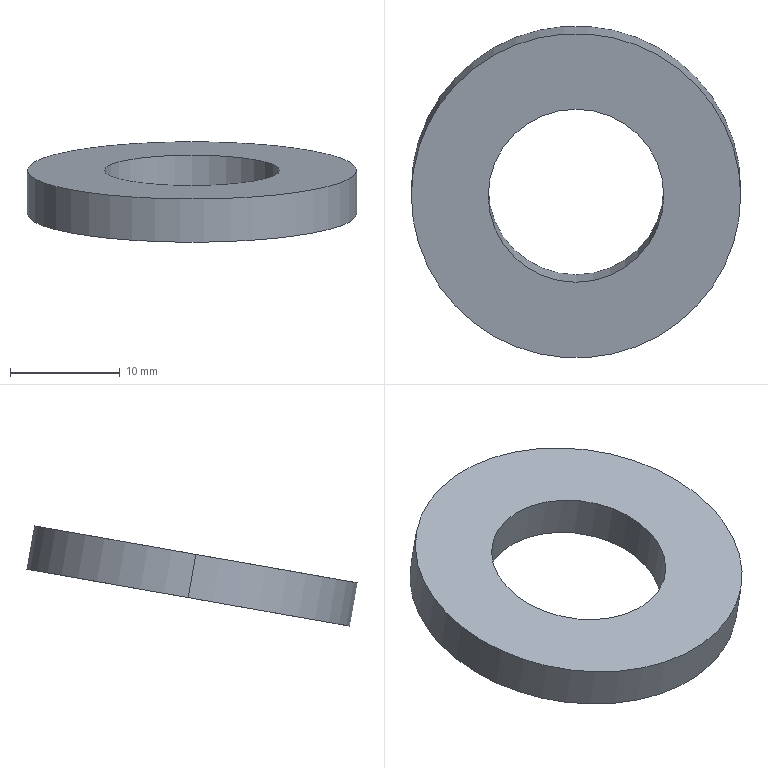Component | SolidWorks | 26Washer-1 | 1 solid | 6 faces | box 30 x 30.24 x 9.15 mm | volume 2023 mm3 | cylinder 4 | plane 2 | commonest cylinder face diameters 16 x2 30 x2
build123d program:
from build123d import *

# Parameters (mm, degrees)
SKETCH1_R           = 15
SKETCH1_R_2         = 8
BOSS_EXTRUDE1_DEPTH = 4


with BuildPart() as part:
    # Sketch1 → Boss-Extrude1 (new body)
    with BuildSketch(Plane.XY):
        Circle(SKETCH1_R)
        Circle(SKETCH1_R_2, mode=Mode.SUBTRACT)
    extrude(amount=BOSS_EXTRUDE1_DEPTH)


solid = part.part

# Placed as in the assembly
solid = solid.moved(Location((79.885, -178.472, 598.663), (10, 0, -14.315)))
STEP:
#1=CARTESIAN_POINT('',(2.83,-7.054,23.725));
#2=VERTEX_POINT('',#1);
#3=CARTESIAN_POINT('',(3.46,-7.054,23.725));
#4=VERTEX_POINT('',#3);
#5=CARTESIAN_POINT('',(3.145,-7.054,23.725));
#6=DIRECTION('',(0.,-0.1736,0.9848));
#7=DIRECTION('',(1.,0.,0.));
#8=AXIS2_PLACEMENT_3D('',#5,#6,#7);
#9=CIRCLE('',#8,0.315);
#10=EDGE_CURVE('',#2,#4,#9,.T.);
#11=ORIENTED_EDGE('',*,*,#10,.T.);
#12=CARTESIAN_POINT('',(3.46,-7.026,23.569));
#13=VERTEX_POINT('',#12);
#14=CARTESIAN_POINT('',(3.46,-7.054,23.725));
#15=DIRECTION('',(0.,0.1736,-0.9848));
#16=VECTOR('',#15,39.37);
#17=LINE('',#14,#16);
#18=EDGE_CURVE('',#4,#13,#17,.T.);
#19=ORIENTED_EDGE('',*,*,#18,.T.);
#20=CARTESIAN_POINT('',(2.83,-7.026,23.569));
#21=VERTEX_POINT('',#20);
#22=CARTESIAN_POINT('',(3.145,-7.026,23.569));
#23=DIRECTION('',(0.,-0.1736,0.9848));
#24=DIRECTION('',(1.,0.,0.));
#25=AXIS2_PLACEMENT_3D('',#22,#23,#24);
#26=CIRCLE('',#25,0.315);
#27=EDGE_CURVE('',#21,#13,#26,.T.);
#28=ORIENTED_EDGE('',*,*,#27,.F.);
#29=CARTESIAN_POINT('',(2.83,-7.054,23.725));
#30=DIRECTION('',(0.,0.1736,-0.9848));
#31=VECTOR('',#30,39.37);
#32=LINE('',#29,#31);
#33=EDGE_CURVE('',#2,#21,#32,.T.);
#34=ORIENTED_EDGE('',*,*,#33,.F.);
#35=EDGE_LOOP('',(#11,#19,#28,#34));
#36=FACE_OUTER_BOUND('',#35,.T.);
#37=CARTESIAN_POINT('',(3.145,-7.054,23.725));
#38=DIRECTION('',(0.,0.1736,-0.9848));
#39=DIRECTION('',(-1.,0.,0.));
#40=AXIS2_PLACEMENT_3D('',#37,#38,#39);
#41=CYLINDRICAL_SURFACE('',#40,0.315);
#42=ADVANCED_FACE('',(#36),#41,.F.);
#43=CARTESIAN_POINT('',(3.736,-7.054,23.725));
#44=VERTEX_POINT('',#43);
#45=CARTESIAN_POINT('',(2.555,-7.054,23.725));
#46=VERTEX_POINT('',#45);
#47=CARTESIAN_POINT('',(3.145,-7.054,23.725));
#48=DIRECTION('',(0.,-0.1736,0.9848));
#49=DIRECTION('',(1.,0.,0.));
#50=AXIS2_PLACEMENT_3D('',#47,#48,#49);
#51=CIRCLE('',#50,0.5906);
#52=EDGE_CURVE('',#44,#46,#51,.T.);
#53=ORIENTED_EDGE('',*,*,#52,.F.);
#54=CARTESIAN_POINT('',(3.736,-7.026,23.569));
#55=VERTEX_POINT('',#54);
#56=CARTESIAN_POINT('',(3.736,-7.054,23.725));
#57=DIRECTION('',(0.,0.1736,-0.9848));
#58=VECTOR('',#57,39.37);
#59=LINE('',#56,#58);
#60=EDGE_CURVE('',#44,#55,#59,.T.);
#61=ORIENTED_EDGE('',*,*,#60,.T.);
#62=CARTESIAN_POINT('',(2.555,-7.026,23.569));
#63=VERTEX_POINT('',#62);
#64=CARTESIAN_POINT('',(3.145,-7.026,23.569));
#65=DIRECTION('',(0.,-0.1736,0.9848));
#66=DIRECTION('',(1.,0.,0.));
#67=AXIS2_PLACEMENT_3D('',#64,#65,#66);
#68=CIRCLE('',#67,0.5906);
#69=EDGE_CURVE('',#55,#63,#68,.T.);
#70=ORIENTED_EDGE('',*,*,#69,.T.);
#71=CARTESIAN_POINT('',(2.555,-7.054,23.725));
#72=DIRECTION('',(0.,0.1736,-0.9848));
#73=VECTOR('',#72,39.37);
#74=LINE('',#71,#73);
#75=EDGE_CURVE('',#46,#63,#74,.T.);
#76=ORIENTED_EDGE('',*,*,#75,.F.);
#77=EDGE_LOOP('',(#53,#61,#70,#76));
#78=FACE_OUTER_BOUND('',#77,.T.);
#79=CARTESIAN_POINT('',(3.145,-7.054,23.725));
#80=DIRECTION('',(0.,0.1736,-0.9848));
#81=DIRECTION('',(-1.,0.,0.));
#82=AXIS2_PLACEMENT_3D('',#79,#80,#81);
#83=CYLINDRICAL_SURFACE('',#82,0.5906);
#84=ADVANCED_FACE('',(#78),#83,.T.);
#85=CARTESIAN_POINT('',(3.145,-7.054,23.725));
#86=DIRECTION('',(0.,-0.1736,0.9848));
#87=DIRECTION('',(1.,0.,0.));
#88=AXIS2_PLACEMENT_3D('',#85,#86,#87);
#89=CIRCLE('',#88,0.5906);
#90=EDGE_CURVE('',#46,#44,#89,.T.);
#91=ORIENTED_EDGE('',*,*,#90,.T.);
#92=ORIENTED_EDGE('',*,*,#52,.T.);
#93=EDGE_LOOP('',(#91,#92));
#94=FACE_OUTER_BOUND('',#93,.T.);
#95=ORIENTED_EDGE('',*,*,#10,.F.);
#96=CARTESIAN_POINT('',(3.145,-7.054,23.725));
#97=DIRECTION('',(0.,-0.1736,0.9848));
#98=DIRECTION('',(1.,0.,0.));
#99=AXIS2_PLACEMENT_3D('',#96,#97,#98);
#100=CIRCLE('',#99,0.315);
#101=EDGE_CURVE('',#4,#2,#100,.T.);
#102=ORIENTED_EDGE('',*,*,#101,.F.);
#103=EDGE_LOOP('',(#95,#102));
#104=FACE_BOUND('',#103,.T.);
#105=CARTESIAN_POINT('',(3.145,-7.054,23.725));
#106=DIRECTION('',(0.,-0.1736,0.9848));
#107=DIRECTION('',(1.,0.,0.));
#108=AXIS2_PLACEMENT_3D('',#105,#106,#107);
#109=PLANE('',#108);
#110=ADVANCED_FACE('',(#94,#104),#109,.T.);
#111=CARTESIAN_POINT('',(3.145,-7.026,23.569));
#112=DIRECTION('',(0.,-0.1736,0.9848));
#113=DIRECTION('',(1.,0.,0.));
#114=AXIS2_PLACEMENT_3D('',#111,#112,#113);
#115=CIRCLE('',#114,0.5906);
#116=EDGE_CURVE('',#63,#55,#115,.T.);
#117=ORIENTED_EDGE('',*,*,#116,.F.);
#118=ORIENTED_EDGE('',*,*,#69,.F.);
#119=EDGE_LOOP('',(#117,#118));
#120=FACE_OUTER_BOUND('',#119,.T.);
#121=ORIENTED_EDGE('',*,*,#27,.T.);
#122=CARTESIAN_POINT('',(3.145,-7.026,23.569));
#123=DIRECTION('',(0.,-0.1736,0.9848));
#124=DIRECTION('',(1.,0.,0.));
#125=AXIS2_PLACEMENT_3D('',#122,#123,#124);
#126=CIRCLE('',#125,0.315);
#127=EDGE_CURVE('',#13,#21,#126,.T.);
#128=ORIENTED_EDGE('',*,*,#127,.T.);
#129=EDGE_LOOP('',(#121,#128));
#130=FACE_BOUND('',#129,.T.);
#131=CARTESIAN_POINT('',(3.145,-7.026,23.569));
#132=DIRECTION('',(0.,-0.1736,0.9848));
#133=DIRECTION('',(1.,0.,0.));
#134=AXIS2_PLACEMENT_3D('',#131,#132,#133);
#135=PLANE('',#134);
#136=ADVANCED_FACE('',(#120,#130),#135,.F.);
#137=ORIENTED_EDGE('',*,*,#60,.F.);
#138=ORIENTED_EDGE('',*,*,#90,.F.);
#139=ORIENTED_EDGE('',*,*,#75,.T.);
#140=ORIENTED_EDGE('',*,*,#116,.T.);
#141=EDGE_LOOP('',(#137,#138,#139,#140));
#142=FACE_OUTER_BOUND('',#141,.T.);
#143=CARTESIAN_POINT('',(3.145,-7.054,23.725));
#144=DIRECTION('',(0.,0.1736,-0.9848));
#145=DIRECTION('',(-1.,0.,0.));
#146=AXIS2_PLACEMENT_3D('',#143,#144,#145);
#147=CYLINDRICAL_SURFACE('',#146,0.5906);
#148=ADVANCED_FACE('',(#142),#147,.T.);
#149=ORIENTED_EDGE('',*,*,#18,.F.);
#150=ORIENTED_EDGE('',*,*,#101,.T.);
#151=ORIENTED_EDGE('',*,*,#33,.T.);
#152=ORIENTED_EDGE('',*,*,#127,.F.);
#153=EDGE_LOOP('',(#149,#150,#151,#152));
#154=FACE_OUTER_BOUND('',#153,.T.);
#155=CARTESIAN_POINT('',(3.145,-7.054,23.725));
#156=DIRECTION('',(0.,0.1736,-0.9848));
#157=DIRECTION('',(-1.,0.,0.));
#158=AXIS2_PLACEMENT_3D('',#155,#156,#157);
#159=CYLINDRICAL_SURFACE('',#158,0.315);
#160=ADVANCED_FACE('',(#154),#159,.F.);
#161=CLOSED_SHELL('',(#42,#84,#110,#136,#148,#160));
#162=MANIFOLD_SOLID_BREP('',#161);
#163=CARTESIAN_POINT('',(0.,0.,0.));
#164=DIRECTION('',(0.,0.,1.));
#165=DIRECTION('',(1.,0.,0.));
#166=AXIS2_PLACEMENT_3D('',#163,#164,#165);
#167=(LENGTH_UNIT()NAMED_UNIT(*)SI_UNIT($,.METRE.));
#168=LENGTH_MEASURE_WITH_UNIT(LENGTH_MEASURE(0.0254),#167);
#169=DIMENSIONAL_EXPONENTS(1.,0.,0.,0.,0.,0.,0.);
#170=(CONVERSION_BASED_UNIT('',#168)LENGTH_UNIT()NAMED_UNIT(#169));
#171=UNCERTAINTY_MEASURE_WITH_UNIT(LENGTH_MEASURE(0.00001),#170,'','');
#172=(NAMED_UNIT(*)PLANE_ANGLE_UNIT()SI_UNIT($,.RADIAN.));
#173=(NAMED_UNIT(*)SI_UNIT($,.STERADIAN.)SOLID_ANGLE_UNIT());
#174=(GEOMETRIC_REPRESENTATION_CONTEXT(3)GLOBAL_UNCERTAINTY_ASSIGNED_CONTEXT((#171))GLOBAL_UNIT_ASSIGNED_CONTEXT((#170,#172,#173))REPRESENTATION_CONTEXT('',''));
#175=ADVANCED_BREP_SHAPE_REPRESENTATION('',(#162,#166),#174);
#176=COLOUR_RGB('',0.7922,0.8196,0.9333);
#177=FILL_AREA_STYLE_COLOUR('',#176);
#178=FILL_AREA_STYLE('',(#177));
#179=SURFACE_STYLE_FILL_AREA(#178);
#180=SURFACE_SIDE_STYLE('',(#179));
#181=SURFACE_STYLE_USAGE(.BOTH.,#180);
#182=PRESENTATION_STYLE_ASSIGNMENT((#181));
#183=STYLED_ITEM('',(#182),#162);
#184=(LENGTH_UNIT()NAMED_UNIT(*)SI_UNIT($,.METRE.));
#185=LENGTH_MEASURE_WITH_UNIT(LENGTH_MEASURE(0.0254),#184);
#186=DIMENSIONAL_EXPONENTS(1.,0.,0.,0.,0.,0.,0.);
#187=(CONVERSION_BASED_UNIT('',#185)LENGTH_UNIT()NAMED_UNIT(#186));
#188=UNCERTAINTY_MEASURE_WITH_UNIT(LENGTH_MEASURE(0.00001),#187,'','');
#189=(NAMED_UNIT(*)PLANE_ANGLE_UNIT()SI_UNIT($,.RADIAN.));
#190=(NAMED_UNIT(*)SI_UNIT($,.STERADIAN.)SOLID_ANGLE_UNIT());
#191=(GEOMETRIC_REPRESENTATION_CONTEXT(3)GLOBAL_UNCERTAINTY_ASSIGNED_CONTEXT((#188))GLOBAL_UNIT_ASSIGNED_CONTEXT((#187,#189,#190))REPRESENTATION_CONTEXT('',''));
#192=MECHANICAL_DESIGN_GEOMETRIC_PRESENTATION_REPRESENTATION('',(#183),#191);
#193=PRESENTATION_LAYER_ASSIGNMENT('','',(#183));